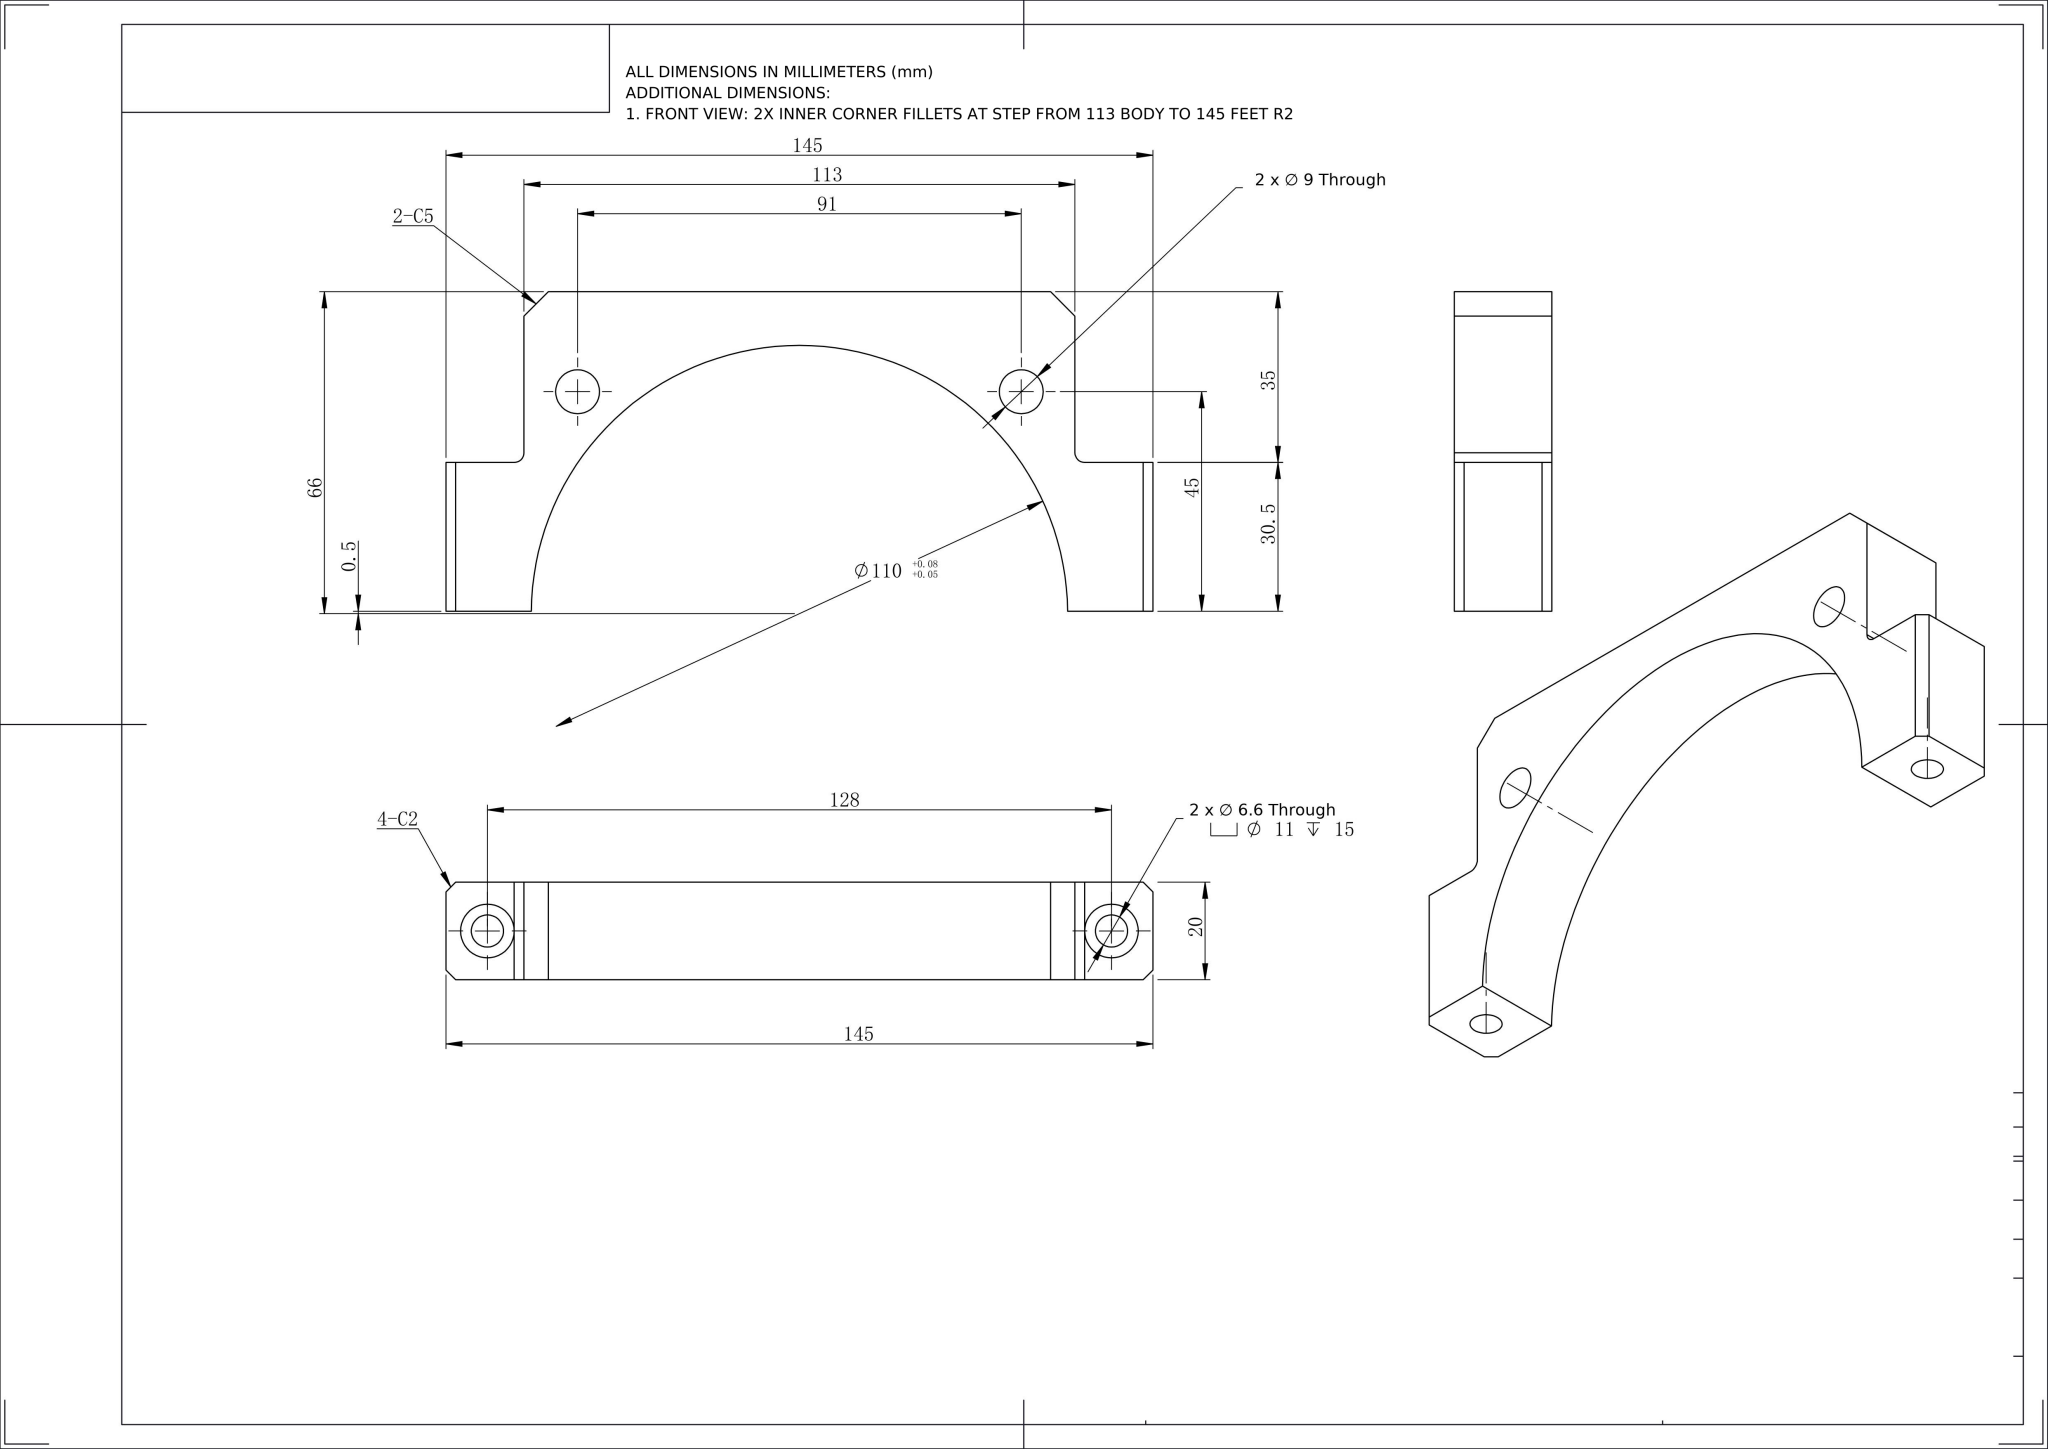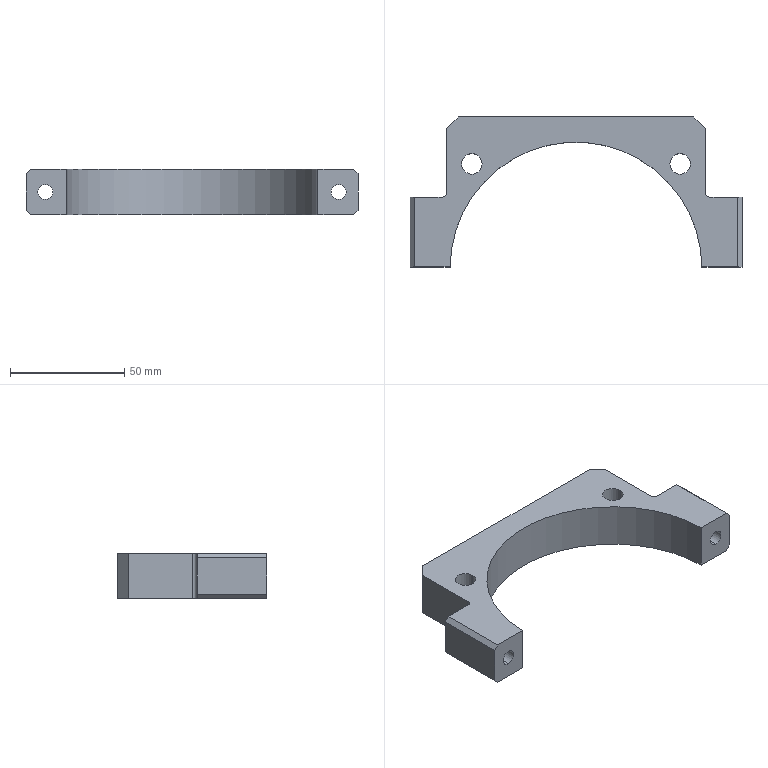Part | NX | mm | 1 solid | 34 faces | box 145 x 65.5 x 20 mm | volume 66451 mm3 | plane 19 | cylinder 15 | commonest cylinder face diameters 9 x4 11 x4 6.6 x4 4 x2 110 x1